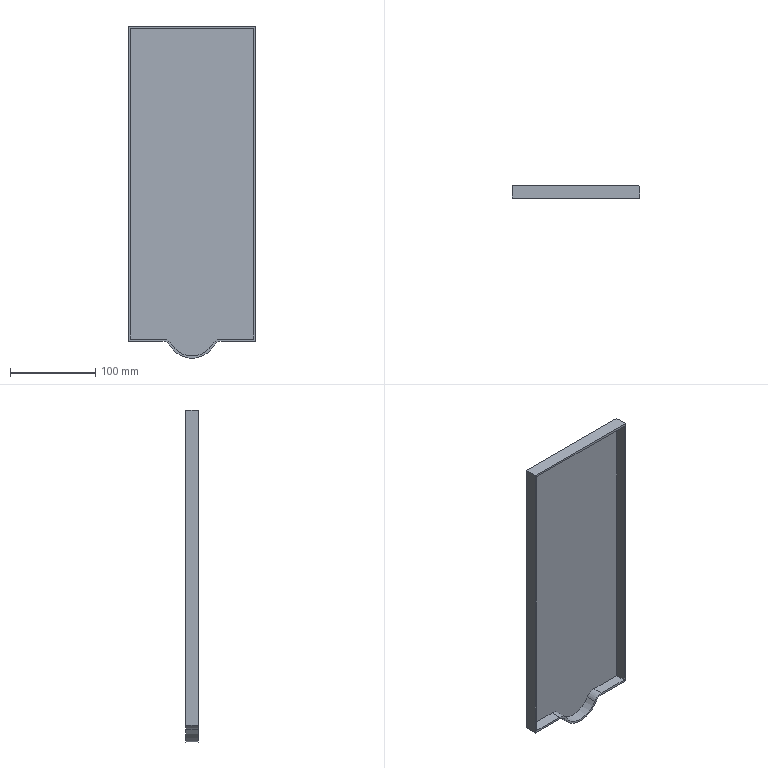Component | SolidWorks | SeedBoxCover-1 | 1 solid | 20 faces | box 150 x 15 x 390 mm | volume 172770 mm3 | plane 13 | cylinder 7 | commonest cylinder face diameters 20 x2 25 x2 60 x1 55 x1 6 x1
build123d program:
from build123d import *

# Parameters (mm, degrees)
SKETCH1_W           = 370
SKETCH1_H           = 150
BOSS_EXTRUDE1_DEPTH = 15
BOSS_EXTRUDE2_DEPTH = 15
FILLET2_R           = 10
SHELL1_T            = -2.5
FILLET3_R           = 3


with BuildPart() as part:
    # Sketch1 → Boss-Extrude1 (new body)
    with BuildSketch(Plane(origin=(0, 0, 0), x_dir=(1, 0, 0), z_dir=(0, 1, 0))):
        Rectangle(SKETCH1_W, SKETCH1_H)
    extrude(amount=BOSS_EXTRUDE1_DEPTH)

    # Sketch3 → Boss-Extrude2 (add)
    with BuildSketch(Plane(origin=(0, 15, 0), x_dir=(1, 0, 0), z_dir=(0, 1, 0))):
        with BuildLine():
            Line((185, 28.284), (185, -28.284))
            ThreePointArc((185, -28.284), (205, 0), (185, 28.284))
        make_face()
    extrude(amount=-BOSS_EXTRUDE2_DEPTH)

    # Fillet2
    fillet2_edges = [part.edges().sort_by_distance(p)[0] for p in [
        (185, 7.5, -28.284),
        (185, 7.5, 28.284),
    ]]
    fillet(fillet2_edges, radius=FILLET2_R)

    # Shell1
    shell1_openings = [part.faces().sort_by_distance(p)[0] for p in [
        (2.873, 0, 0),
    ]]
    offset(amount=SHELL1_T, openings=shell1_openings, kind=Kind.INTERSECTION)

    # Fillet3
    fillet3_edges = [part.edges().sort_by_distance(p)[0] for p in [
        (0, 15, 75),
    ]]
    fillet(fillet3_edges, radius=FILLET3_R)


solid = part.part

# Placed as in the assembly
solid = solid.moved(Location((-5.5, 550, -326.036), (0, 90, 0)))
STEP:
#1=COLOUR_RGB('',0.7922,0.8196,0.9333);
#2=FILL_AREA_STYLE_COLOUR('',#1);
#3=FILL_AREA_STYLE('',(#2));
#4=SURFACE_STYLE_FILL_AREA(#3);
#5=SURFACE_SIDE_STYLE('',(#4));
#6=SURFACE_STYLE_USAGE(.BOTH.,#5);
#7=PRESENTATION_STYLE_ASSIGNMENT((#6));
#8=CARTESIAN_POINT('',(2.736,21.654,-20.12));
#9=VERTEX_POINT('',#8);
#10=CARTESIAN_POINT('',(1.147,21.654,-20.12));
#11=VERTEX_POINT('',#10);
#12=CARTESIAN_POINT('',(2.736,21.654,-20.12));
#13=DIRECTION('',(-1.,-0.,0.));
#14=VECTOR('',#13,39.37);
#15=LINE('',#12,#14);
#16=EDGE_CURVE('',#9,#11,#15,.T.);
#17=ORIENTED_EDGE('',*,*,#16,.F.);
#18=CARTESIAN_POINT('',(2.736,21.654,-5.553));
#19=VERTEX_POINT('',#18);
#20=CARTESIAN_POINT('',(2.736,21.654,-5.553));
#21=DIRECTION('',(-0.,0.,-1.));
#22=VECTOR('',#21,39.37);
#23=LINE('',#20,#22);
#24=EDGE_CURVE('',#19,#9,#23,.T.);
#25=ORIENTED_EDGE('',*,*,#24,.F.);
#26=CARTESIAN_POINT('',(-3.169,21.654,-5.553));
#27=VERTEX_POINT('',#26);
#28=CARTESIAN_POINT('',(2.736,21.654,-5.553));
#29=DIRECTION('',(1.,0.,-0.));
#30=VECTOR('',#29,39.37);
#31=LINE('',#28,#30);
#32=EDGE_CURVE('',#27,#19,#31,.T.);
#33=ORIENTED_EDGE('',*,*,#32,.F.);
#34=CARTESIAN_POINT('',(-3.169,21.654,-20.12));
#35=VERTEX_POINT('',#34);
#36=CARTESIAN_POINT('',(-3.169,21.654,-5.553));
#37=DIRECTION('',(0.,-0.,1.));
#38=VECTOR('',#37,39.37);
#39=LINE('',#36,#38);
#40=EDGE_CURVE('',#35,#27,#39,.T.);
#41=ORIENTED_EDGE('',*,*,#40,.F.);
#42=CARTESIAN_POINT('',(-1.58,21.654,-20.12));
#43=VERTEX_POINT('',#42);
#44=CARTESIAN_POINT('',(2.736,21.654,-20.12));
#45=DIRECTION('',(-1.,-0.,0.));
#46=VECTOR('',#45,39.37);
#47=LINE('',#44,#46);
#48=EDGE_CURVE('',#43,#35,#47,.T.);
#49=ORIENTED_EDGE('',*,*,#48,.F.);
#50=CARTESIAN_POINT('',(-1.239,21.654,-20.316));
#51=VERTEX_POINT('',#50);
#52=CARTESIAN_POINT('',(-1.58,21.654,-20.513));
#53=DIRECTION('',(-0.,1.,0.));
#54=DIRECTION('',(-1.,0.,0.));
#55=AXIS2_PLACEMENT_3D('',#52,#53,#54);
#56=CIRCLE('',#55,0.3937);
#57=EDGE_CURVE('',#43,#51,#56,.T.);
#58=ORIENTED_EDGE('',*,*,#57,.T.);
#59=CARTESIAN_POINT('',(0.8063,21.654,-20.316));
#60=VERTEX_POINT('',#59);
#61=CARTESIAN_POINT('',(-0.2165,21.654,-19.726));
#62=DIRECTION('',(-0.,1.,0.));
#63=DIRECTION('',(-1.,0.,0.));
#64=AXIS2_PLACEMENT_3D('',#61,#62,#63);
#65=CIRCLE('',#64,1.181);
#66=EDGE_CURVE('',#60,#51,#65,.T.);
#67=ORIENTED_EDGE('',*,*,#66,.F.);
#68=CARTESIAN_POINT('',(1.147,21.654,-20.513));
#69=DIRECTION('',(-0.,1.,0.));
#70=DIRECTION('',(-1.,0.,0.));
#71=AXIS2_PLACEMENT_3D('',#68,#69,#70);
#72=CIRCLE('',#71,0.3937);
#73=EDGE_CURVE('',#60,#11,#72,.T.);
#74=ORIENTED_EDGE('',*,*,#73,.T.);
#75=EDGE_LOOP('',(#17,#25,#33,#41,#49,#58,#67,#74));
#76=FACE_OUTER_BOUND('',#75,.T.);
#77=CARTESIAN_POINT('',(2.638,21.654,-5.651));
#78=VERTEX_POINT('',#77);
#79=CARTESIAN_POINT('',(2.638,21.654,-20.021));
#80=VERTEX_POINT('',#79);
#81=CARTESIAN_POINT('',(2.638,21.654,-12.836));
#82=DIRECTION('',(-0.,0.,-1.));
#83=VECTOR('',#82,39.37);
#84=LINE('',#81,#83);
#85=EDGE_CURVE('',#78,#80,#84,.T.);
#86=ORIENTED_EDGE('',*,*,#85,.T.);
#87=CARTESIAN_POINT('',(1.147,21.654,-20.021));
#88=VERTEX_POINT('',#87);
#89=CARTESIAN_POINT('',(-0.2165,21.654,-20.021));
#90=DIRECTION('',(-1.,-0.,0.));
#91=VECTOR('',#90,39.37);
#92=LINE('',#89,#91);
#93=EDGE_CURVE('',#80,#88,#92,.T.);
#94=ORIENTED_EDGE('',*,*,#93,.T.);
#95=CARTESIAN_POINT('',(0.7211,21.654,-20.267));
#96=VERTEX_POINT('',#95);
#97=CARTESIAN_POINT('',(1.147,21.654,-20.513));
#98=DIRECTION('',(-0.,1.,0.));
#99=DIRECTION('',(-1.,0.,0.));
#100=AXIS2_PLACEMENT_3D('',#97,#98,#99);
#101=CIRCLE('',#100,0.4921);
#102=EDGE_CURVE('',#96,#88,#101,.T.);
#103=ORIENTED_EDGE('',*,*,#102,.F.);
#104=CARTESIAN_POINT('',(-1.154,21.654,-20.267));
#105=VERTEX_POINT('',#104);
#106=CARTESIAN_POINT('',(-0.2165,21.654,-19.726));
#107=DIRECTION('',(-0.,1.,0.));
#108=DIRECTION('',(-1.,0.,-0.));
#109=AXIS2_PLACEMENT_3D('',#106,#107,#108);
#110=CIRCLE('',#109,1.083);
#111=EDGE_CURVE('',#96,#105,#110,.T.);
#112=ORIENTED_EDGE('',*,*,#111,.T.);
#113=CARTESIAN_POINT('',(-1.58,21.654,-20.021));
#114=VERTEX_POINT('',#113);
#115=CARTESIAN_POINT('',(-1.58,21.654,-20.513));
#116=DIRECTION('',(-0.,1.,0.));
#117=DIRECTION('',(-1.,0.,0.));
#118=AXIS2_PLACEMENT_3D('',#115,#116,#117);
#119=CIRCLE('',#118,0.4921);
#120=EDGE_CURVE('',#114,#105,#119,.T.);
#121=ORIENTED_EDGE('',*,*,#120,.F.);
#122=CARTESIAN_POINT('',(-3.071,21.654,-20.021));
#123=VERTEX_POINT('',#122);
#124=CARTESIAN_POINT('',(-0.2165,21.654,-20.021));
#125=DIRECTION('',(-1.,-0.,0.));
#126=VECTOR('',#125,39.37);
#127=LINE('',#124,#126);
#128=EDGE_CURVE('',#114,#123,#127,.T.);
#129=ORIENTED_EDGE('',*,*,#128,.T.);
#130=CARTESIAN_POINT('',(-3.071,21.654,-5.651));
#131=VERTEX_POINT('',#130);
#132=CARTESIAN_POINT('',(-3.071,21.654,-12.836));
#133=DIRECTION('',(0.,-0.,1.));
#134=VECTOR('',#133,39.37);
#135=LINE('',#132,#134);
#136=EDGE_CURVE('',#123,#131,#135,.T.);
#137=ORIENTED_EDGE('',*,*,#136,.T.);
#138=CARTESIAN_POINT('',(-0.2165,21.654,-5.651));
#139=DIRECTION('',(1.,0.,-0.));
#140=VECTOR('',#139,39.37);
#141=LINE('',#138,#140);
#142=EDGE_CURVE('',#131,#78,#141,.T.);
#143=ORIENTED_EDGE('',*,*,#142,.T.);
#144=EDGE_LOOP('',(#86,#94,#103,#112,#121,#129,#137,#143));
#145=FACE_BOUND('',#144,.T.);
#146=CARTESIAN_POINT('',(-0.2165,21.654,-12.836));
#147=DIRECTION('',(0.,-1.,-0.));
#148=DIRECTION('',(-1.,-0.,0.));
#149=AXIS2_PLACEMENT_3D('',#146,#147,#148);
#150=PLANE('',#149);
#151=ADVANCED_FACE('',(#76,#145),#150,.T.);
#152=CARTESIAN_POINT('',(2.618,22.244,-20.12));
#153=VERTEX_POINT('',#152);
#154=CARTESIAN_POINT('',(1.147,22.244,-20.12));
#155=VERTEX_POINT('',#154);
#156=CARTESIAN_POINT('',(2.736,22.244,-20.12));
#157=DIRECTION('',(-1.,-0.,0.));
#158=VECTOR('',#157,39.37);
#159=LINE('',#156,#158);
#160=EDGE_CURVE('',#153,#155,#159,.T.);
#161=ORIENTED_EDGE('',*,*,#160,.F.);
#162=CARTESIAN_POINT('',(2.736,22.126,-20.12));
#163=VERTEX_POINT('',#162);
#164=CARTESIAN_POINT('',(2.618,22.126,-20.12));
#165=DIRECTION('',(-0.,0.,-1.));
#166=DIRECTION('',(1.,0.,0.));
#167=AXIS2_PLACEMENT_3D('',#164,#165,#166);
#168=CIRCLE('',#167,0.1181);
#169=EDGE_CURVE('',#153,#163,#168,.T.);
#170=ORIENTED_EDGE('',*,*,#169,.T.);
#171=CARTESIAN_POINT('',(2.736,22.244,-20.12));
#172=DIRECTION('',(0.,-1.,-0.));
#173=VECTOR('',#172,39.37);
#174=LINE('',#171,#173);
#175=EDGE_CURVE('',#163,#9,#174,.T.);
#176=ORIENTED_EDGE('',*,*,#175,.T.);
#177=ORIENTED_EDGE('',*,*,#16,.T.);
#178=CARTESIAN_POINT('',(1.147,22.244,-20.12));
#179=DIRECTION('',(-0.,1.,0.));
#180=VECTOR('',#179,39.37);
#181=LINE('',#178,#180);
#182=EDGE_CURVE('',#11,#155,#181,.T.);
#183=ORIENTED_EDGE('',*,*,#182,.T.);
#184=EDGE_LOOP('',(#161,#170,#176,#177,#183));
#185=FACE_OUTER_BOUND('',#184,.T.);
#186=CARTESIAN_POINT('',(2.736,22.244,-20.12));
#187=DIRECTION('',(0.,-0.,1.));
#188=DIRECTION('',(1.,0.,-0.));
#189=AXIS2_PLACEMENT_3D('',#186,#187,#188);
#190=PLANE('',#189);
#191=ADVANCED_FACE('',(#185),#190,.F.);
#192=CARTESIAN_POINT('',(-1.58,22.244,-20.12));
#193=VERTEX_POINT('',#192);
#194=CARTESIAN_POINT('',(-3.169,22.244,-20.12));
#195=VERTEX_POINT('',#194);
#196=CARTESIAN_POINT('',(2.736,22.244,-20.12));
#197=DIRECTION('',(-1.,-0.,0.));
#198=VECTOR('',#197,39.37);
#199=LINE('',#196,#198);
#200=EDGE_CURVE('',#193,#195,#199,.T.);
#201=ORIENTED_EDGE('',*,*,#200,.F.);
#202=CARTESIAN_POINT('',(-1.58,22.244,-20.12));
#203=DIRECTION('',(0.,-1.,-0.));
#204=VECTOR('',#203,39.37);
#205=LINE('',#202,#204);
#206=EDGE_CURVE('',#193,#43,#205,.T.);
#207=ORIENTED_EDGE('',*,*,#206,.T.);
#208=ORIENTED_EDGE('',*,*,#48,.T.);
#209=CARTESIAN_POINT('',(-3.169,22.244,-20.12));
#210=DIRECTION('',(0.,-1.,-0.));
#211=VECTOR('',#210,39.37);
#212=LINE('',#209,#211);
#213=EDGE_CURVE('',#195,#35,#212,.T.);
#214=ORIENTED_EDGE('',*,*,#213,.F.);
#215=EDGE_LOOP('',(#201,#207,#208,#214));
#216=FACE_OUTER_BOUND('',#215,.T.);
#217=CARTESIAN_POINT('',(2.736,22.244,-20.12));
#218=DIRECTION('',(0.,-0.,1.));
#219=DIRECTION('',(1.,0.,-0.));
#220=AXIS2_PLACEMENT_3D('',#217,#218,#219);
#221=PLANE('',#220);
#222=ADVANCED_FACE('',(#216),#221,.F.);
#223=ORIENTED_EDGE('',*,*,#40,.T.);
#224=CARTESIAN_POINT('',(-3.169,22.244,-5.553));
#225=VERTEX_POINT('',#224);
#226=CARTESIAN_POINT('',(-3.169,22.244,-5.553));
#227=DIRECTION('',(0.,-1.,-0.));
#228=VECTOR('',#227,39.37);
#229=LINE('',#226,#228);
#230=EDGE_CURVE('',#225,#27,#229,.T.);
#231=ORIENTED_EDGE('',*,*,#230,.F.);
#232=CARTESIAN_POINT('',(-3.169,22.244,-5.553));
#233=DIRECTION('',(0.,-0.,1.));
#234=VECTOR('',#233,39.37);
#235=LINE('',#232,#234);
#236=EDGE_CURVE('',#195,#225,#235,.T.);
#237=ORIENTED_EDGE('',*,*,#236,.F.);
#238=ORIENTED_EDGE('',*,*,#213,.T.);
#239=EDGE_LOOP('',(#223,#231,#237,#238));
#240=FACE_OUTER_BOUND('',#239,.T.);
#241=CARTESIAN_POINT('',(-3.169,22.244,-5.553));
#242=DIRECTION('',(1.,0.,-0.));
#243=DIRECTION('',(-0.,0.,-1.));
#244=AXIS2_PLACEMENT_3D('',#241,#242,#243);
#245=PLANE('',#244);
#246=ADVANCED_FACE('',(#240),#245,.F.);
#247=CARTESIAN_POINT('',(2.736,22.126,-5.553));
#248=VERTEX_POINT('',#247);
#249=CARTESIAN_POINT('',(2.736,22.244,-5.553));
#250=DIRECTION('',(0.,-1.,-0.));
#251=VECTOR('',#250,39.37);
#252=LINE('',#249,#251);
#253=EDGE_CURVE('',#248,#19,#252,.T.);
#254=ORIENTED_EDGE('',*,*,#253,.F.);
#255=CARTESIAN_POINT('',(2.618,22.244,-5.553));
#256=VERTEX_POINT('',#255);
#257=CARTESIAN_POINT('',(2.618,22.126,-5.553));
#258=DIRECTION('',(0.,-0.,1.));
#259=DIRECTION('',(-1.,0.,0.));
#260=AXIS2_PLACEMENT_3D('',#257,#258,#259);
#261=CIRCLE('',#260,0.1181);
#262=EDGE_CURVE('',#248,#256,#261,.T.);
#263=ORIENTED_EDGE('',*,*,#262,.T.);
#264=CARTESIAN_POINT('',(2.736,22.244,-5.553));
#265=DIRECTION('',(1.,0.,-0.));
#266=VECTOR('',#265,39.37);
#267=LINE('',#264,#266);
#268=EDGE_CURVE('',#225,#256,#267,.T.);
#269=ORIENTED_EDGE('',*,*,#268,.F.);
#270=ORIENTED_EDGE('',*,*,#230,.T.);
#271=ORIENTED_EDGE('',*,*,#32,.T.);
#272=EDGE_LOOP('',(#254,#263,#269,#270,#271));
#273=FACE_OUTER_BOUND('',#272,.T.);
#274=CARTESIAN_POINT('',(2.736,22.244,-5.553));
#275=DIRECTION('',(-0.,0.,-1.));
#276=DIRECTION('',(-1.,-0.,0.));
#277=AXIS2_PLACEMENT_3D('',#274,#275,#276);
#278=PLANE('',#277);
#279=ADVANCED_FACE('',(#273),#278,.F.);
#280=ORIENTED_EDGE('',*,*,#175,.F.);
#281=CARTESIAN_POINT('',(2.736,22.126,-5.553));
#282=DIRECTION('',(0.,-0.,1.));
#283=VECTOR('',#282,39.37);
#284=LINE('',#281,#283);
#285=EDGE_CURVE('',#163,#248,#284,.T.);
#286=ORIENTED_EDGE('',*,*,#285,.T.);
#287=ORIENTED_EDGE('',*,*,#253,.T.);
#288=ORIENTED_EDGE('',*,*,#24,.T.);
#289=EDGE_LOOP('',(#280,#286,#287,#288));
#290=FACE_OUTER_BOUND('',#289,.T.);
#291=CARTESIAN_POINT('',(2.736,22.244,-5.553));
#292=DIRECTION('',(-1.,-0.,0.));
#293=DIRECTION('',(0.,-0.,1.));
#294=AXIS2_PLACEMENT_3D('',#291,#292,#293);
#295=PLANE('',#294);
#296=ADVANCED_FACE('',(#290),#295,.F.);
#297=ORIENTED_EDGE('',*,*,#268,.T.);
#298=CARTESIAN_POINT('',(2.618,22.244,-12.836));
#299=DIRECTION('',(-0.,0.,-1.));
#300=VECTOR('',#299,39.37);
#301=LINE('',#298,#300);
#302=EDGE_CURVE('',#256,#153,#301,.T.);
#303=ORIENTED_EDGE('',*,*,#302,.T.);
#304=ORIENTED_EDGE('',*,*,#160,.T.);
#305=CARTESIAN_POINT('',(0.8063,22.244,-20.316));
#306=VERTEX_POINT('',#305);
#307=CARTESIAN_POINT('',(1.147,22.244,-20.513));
#308=DIRECTION('',(0.,-1.,-0.));
#309=DIRECTION('',(-1.,0.,0.));
#310=AXIS2_PLACEMENT_3D('',#307,#308,#309);
#311=CIRCLE('',#310,0.3937);
#312=EDGE_CURVE('',#155,#306,#311,.T.);
#313=ORIENTED_EDGE('',*,*,#312,.T.);
#314=CARTESIAN_POINT('',(-1.239,22.244,-20.316));
#315=VERTEX_POINT('',#314);
#316=CARTESIAN_POINT('',(-0.2165,22.244,-19.726));
#317=DIRECTION('',(-0.,1.,0.));
#318=DIRECTION('',(-1.,0.,0.));
#319=AXIS2_PLACEMENT_3D('',#316,#317,#318);
#320=CIRCLE('',#319,1.181);
#321=EDGE_CURVE('',#306,#315,#320,.T.);
#322=ORIENTED_EDGE('',*,*,#321,.T.);
#323=CARTESIAN_POINT('',(-1.58,22.244,-20.513));
#324=DIRECTION('',(0.,-1.,-0.));
#325=DIRECTION('',(-1.,0.,0.));
#326=AXIS2_PLACEMENT_3D('',#323,#324,#325);
#327=CIRCLE('',#326,0.3937);
#328=EDGE_CURVE('',#315,#193,#327,.T.);
#329=ORIENTED_EDGE('',*,*,#328,.T.);
#330=ORIENTED_EDGE('',*,*,#200,.T.);
#331=ORIENTED_EDGE('',*,*,#236,.T.);
#332=EDGE_LOOP('',(#297,#303,#304,#313,#322,#329,#330,#331));
#333=FACE_OUTER_BOUND('',#332,.T.);
#334=CARTESIAN_POINT('',(-0.2165,22.244,-12.836));
#335=DIRECTION('',(0.,-1.,-0.));
#336=DIRECTION('',(-1.,-0.,0.));
#337=AXIS2_PLACEMENT_3D('',#334,#335,#336);
#338=PLANE('',#337);
#339=ADVANCED_FACE('',(#333),#338,.F.);
#340=ORIENTED_EDGE('',*,*,#321,.F.);
#341=CARTESIAN_POINT('',(0.8063,21.654,-20.316));
#342=DIRECTION('',(0.,-1.,-0.));
#343=VECTOR('',#342,39.37);
#344=LINE('',#341,#343);
#345=EDGE_CURVE('',#306,#60,#344,.T.);
#346=ORIENTED_EDGE('',*,*,#345,.T.);
#347=ORIENTED_EDGE('',*,*,#66,.T.);
#348=CARTESIAN_POINT('',(-1.239,21.654,-20.316));
#349=DIRECTION('',(-0.,1.,0.));
#350=VECTOR('',#349,39.37);
#351=LINE('',#348,#350);
#352=EDGE_CURVE('',#51,#315,#351,.T.);
#353=ORIENTED_EDGE('',*,*,#352,.T.);
#354=EDGE_LOOP('',(#340,#346,#347,#353));
#355=FACE_OUTER_BOUND('',#354,.T.);
#356=CARTESIAN_POINT('',(-0.2165,21.654,-19.726));
#357=DIRECTION('',(-0.,1.,0.));
#358=DIRECTION('',(1.,0.,0.));
#359=AXIS2_PLACEMENT_3D('',#356,#357,#358);
#360=CYLINDRICAL_SURFACE('',#359,1.181);
#361=ADVANCED_FACE('',(#355),#360,.T.);
#362=ORIENTED_EDGE('',*,*,#73,.F.);
#363=ORIENTED_EDGE('',*,*,#345,.F.);
#364=ORIENTED_EDGE('',*,*,#312,.F.);
#365=ORIENTED_EDGE('',*,*,#182,.F.);
#366=EDGE_LOOP('',(#362,#363,#364,#365));
#367=FACE_OUTER_BOUND('',#366,.T.);
#368=CARTESIAN_POINT('',(1.147,21.654,-20.513));
#369=DIRECTION('',(-0.,1.,0.));
#370=DIRECTION('',(1.,0.,0.));
#371=AXIS2_PLACEMENT_3D('',#368,#369,#370);
#372=CYLINDRICAL_SURFACE('',#371,0.3937);
#373=ADVANCED_FACE('',(#367),#372,.F.);
#374=ORIENTED_EDGE('',*,*,#57,.F.);
#375=ORIENTED_EDGE('',*,*,#206,.F.);
#376=ORIENTED_EDGE('',*,*,#328,.F.);
#377=ORIENTED_EDGE('',*,*,#352,.F.);
#378=EDGE_LOOP('',(#374,#375,#376,#377));
#379=FACE_OUTER_BOUND('',#378,.T.);
#380=CARTESIAN_POINT('',(-1.58,21.654,-20.513));
#381=DIRECTION('',(-0.,1.,0.));
#382=DIRECTION('',(1.,0.,0.));
#383=AXIS2_PLACEMENT_3D('',#380,#381,#382);
#384=CYLINDRICAL_SURFACE('',#383,0.3937);
#385=ADVANCED_FACE('',(#379),#384,.F.);
#386=ORIENTED_EDGE('',*,*,#93,.F.);
#387=CARTESIAN_POINT('',(2.638,22.146,-20.021));
#388=VERTEX_POINT('',#387);
#389=CARTESIAN_POINT('',(2.638,22.244,-20.021));
#390=DIRECTION('',(0.,-1.,-0.));
#391=VECTOR('',#390,39.37);
#392=LINE('',#389,#391);
#393=EDGE_CURVE('',#388,#80,#392,.T.);
#394=ORIENTED_EDGE('',*,*,#393,.F.);
#395=CARTESIAN_POINT('',(1.147,22.146,-20.021));
#396=VERTEX_POINT('',#395);
#397=CARTESIAN_POINT('',(-0.2165,22.146,-20.021));
#398=DIRECTION('',(-1.,-0.,0.));
#399=VECTOR('',#398,39.37);
#400=LINE('',#397,#399);
#401=EDGE_CURVE('',#388,#396,#400,.T.);
#402=ORIENTED_EDGE('',*,*,#401,.T.);
#403=CARTESIAN_POINT('',(1.147,22.244,-20.021));
#404=DIRECTION('',(-0.,1.,0.));
#405=VECTOR('',#404,39.37);
#406=LINE('',#403,#405);
#407=EDGE_CURVE('',#88,#396,#406,.T.);
#408=ORIENTED_EDGE('',*,*,#407,.F.);
#409=EDGE_LOOP('',(#386,#394,#402,#408));
#410=FACE_OUTER_BOUND('',#409,.T.);
#411=CARTESIAN_POINT('',(2.736,22.244,-20.021));
#412=DIRECTION('',(0.,-0.,1.));
#413=DIRECTION('',(1.,0.,-0.));
#414=AXIS2_PLACEMENT_3D('',#411,#412,#413);
#415=PLANE('',#414);
#416=ADVANCED_FACE('',(#410),#415,.T.);
#417=CARTESIAN_POINT('',(-1.58,22.146,-20.021));
#418=VERTEX_POINT('',#417);
#419=CARTESIAN_POINT('',(-3.071,22.146,-20.021));
#420=VERTEX_POINT('',#419);
#421=CARTESIAN_POINT('',(-0.2165,22.146,-20.021));
#422=DIRECTION('',(-1.,-0.,0.));
#423=VECTOR('',#422,39.37);
#424=LINE('',#421,#423);
#425=EDGE_CURVE('',#418,#420,#424,.T.);
#426=ORIENTED_EDGE('',*,*,#425,.T.);
#427=CARTESIAN_POINT('',(-3.071,22.244,-20.021));
#428=DIRECTION('',(0.,-1.,-0.));
#429=VECTOR('',#428,39.37);
#430=LINE('',#427,#429);
#431=EDGE_CURVE('',#420,#123,#430,.T.);
#432=ORIENTED_EDGE('',*,*,#431,.T.);
#433=ORIENTED_EDGE('',*,*,#128,.F.);
#434=CARTESIAN_POINT('',(-1.58,22.244,-20.021));
#435=DIRECTION('',(0.,-1.,-0.));
#436=VECTOR('',#435,39.37);
#437=LINE('',#434,#436);
#438=EDGE_CURVE('',#418,#114,#437,.T.);
#439=ORIENTED_EDGE('',*,*,#438,.F.);
#440=EDGE_LOOP('',(#426,#432,#433,#439));
#441=FACE_OUTER_BOUND('',#440,.T.);
#442=CARTESIAN_POINT('',(2.736,22.244,-20.021));
#443=DIRECTION('',(0.,-0.,1.));
#444=DIRECTION('',(1.,0.,-0.));
#445=AXIS2_PLACEMENT_3D('',#442,#443,#444);
#446=PLANE('',#445);
#447=ADVANCED_FACE('',(#441),#446,.T.);
#448=ORIENTED_EDGE('',*,*,#136,.F.);
#449=ORIENTED_EDGE('',*,*,#431,.F.);
#450=CARTESIAN_POINT('',(-3.071,22.146,-5.651));
#451=VERTEX_POINT('',#450);
#452=CARTESIAN_POINT('',(-3.071,22.146,-12.836));
#453=DIRECTION('',(0.,-0.,1.));
#454=VECTOR('',#453,39.37);
#455=LINE('',#452,#454);
#456=EDGE_CURVE('',#420,#451,#455,.T.);
#457=ORIENTED_EDGE('',*,*,#456,.T.);
#458=CARTESIAN_POINT('',(-3.071,22.244,-5.651));
#459=DIRECTION('',(0.,-1.,-0.));
#460=VECTOR('',#459,39.37);
#461=LINE('',#458,#460);
#462=EDGE_CURVE('',#451,#131,#461,.T.);
#463=ORIENTED_EDGE('',*,*,#462,.T.);
#464=EDGE_LOOP('',(#448,#449,#457,#463));
#465=FACE_OUTER_BOUND('',#464,.T.);
#466=CARTESIAN_POINT('',(-3.071,22.244,-5.553));
#467=DIRECTION('',(1.,0.,-0.));
#468=DIRECTION('',(-0.,0.,-1.));
#469=AXIS2_PLACEMENT_3D('',#466,#467,#468);
#470=PLANE('',#469);
#471=ADVANCED_FACE('',(#465),#470,.T.);
#472=ORIENTED_EDGE('',*,*,#142,.F.);
#473=ORIENTED_EDGE('',*,*,#462,.F.);
#474=CARTESIAN_POINT('',(2.638,22.146,-5.651));
#475=VERTEX_POINT('',#474);
#476=CARTESIAN_POINT('',(-0.2165,22.146,-5.651));
#477=DIRECTION('',(1.,0.,-0.));
#478=VECTOR('',#477,39.37);
#479=LINE('',#476,#478);
#480=EDGE_CURVE('',#451,#475,#479,.T.);
#481=ORIENTED_EDGE('',*,*,#480,.T.);
#482=CARTESIAN_POINT('',(2.638,22.244,-5.651));
#483=DIRECTION('',(0.,-1.,-0.));
#484=VECTOR('',#483,39.37);
#485=LINE('',#482,#484);
#486=EDGE_CURVE('',#475,#78,#485,.T.);
#487=ORIENTED_EDGE('',*,*,#486,.T.);
#488=EDGE_LOOP('',(#472,#473,#481,#487));
#489=FACE_OUTER_BOUND('',#488,.T.);
#490=CARTESIAN_POINT('',(2.736,22.244,-5.651));
#491=DIRECTION('',(-0.,0.,-1.));
#492=DIRECTION('',(-1.,-0.,0.));
#493=AXIS2_PLACEMENT_3D('',#490,#491,#492);
#494=PLANE('',#493);
#495=ADVANCED_FACE('',(#489),#494,.T.);
#496=ORIENTED_EDGE('',*,*,#85,.F.);
#497=ORIENTED_EDGE('',*,*,#486,.F.);
#498=CARTESIAN_POINT('',(2.638,22.146,-12.836));
#499=DIRECTION('',(-0.,0.,-1.));
#500=VECTOR('',#499,39.37);
#501=LINE('',#498,#500);
#502=EDGE_CURVE('',#475,#388,#501,.T.);
#503=ORIENTED_EDGE('',*,*,#502,.T.);
#504=ORIENTED_EDGE('',*,*,#393,.T.);
#505=EDGE_LOOP('',(#496,#497,#503,#504));
#506=FACE_OUTER_BOUND('',#505,.T.);
#507=CARTESIAN_POINT('',(2.638,22.244,-5.553));
#508=DIRECTION('',(-1.,-0.,0.));
#509=DIRECTION('',(0.,-0.,1.));
#510=AXIS2_PLACEMENT_3D('',#507,#508,#509);
#511=PLANE('',#510);
#512=ADVANCED_FACE('',(#506),#511,.T.);
#513=ORIENTED_EDGE('',*,*,#401,.F.);
#514=ORIENTED_EDGE('',*,*,#502,.F.);
#515=ORIENTED_EDGE('',*,*,#480,.F.);
#516=ORIENTED_EDGE('',*,*,#456,.F.);
#517=ORIENTED_EDGE('',*,*,#425,.F.);
#518=CARTESIAN_POINT('',(-1.154,22.146,-20.267));
#519=VERTEX_POINT('',#518);
#520=CARTESIAN_POINT('',(-1.58,22.146,-20.513));
#521=DIRECTION('',(0.,-1.,-0.));
#522=DIRECTION('',(-1.,0.,0.));
#523=AXIS2_PLACEMENT_3D('',#520,#521,#522);
#524=CIRCLE('',#523,0.4921);
#525=EDGE_CURVE('',#519,#418,#524,.T.);
#526=ORIENTED_EDGE('',*,*,#525,.F.);
#527=CARTESIAN_POINT('',(0.7211,22.146,-20.267));
#528=VERTEX_POINT('',#527);
#529=CARTESIAN_POINT('',(-0.2165,22.146,-19.726));
#530=DIRECTION('',(-0.,1.,0.));
#531=DIRECTION('',(-1.,0.,-0.));
#532=AXIS2_PLACEMENT_3D('',#529,#530,#531);
#533=CIRCLE('',#532,1.083);
#534=EDGE_CURVE('',#528,#519,#533,.T.);
#535=ORIENTED_EDGE('',*,*,#534,.F.);
#536=CARTESIAN_POINT('',(1.147,22.146,-20.513));
#537=DIRECTION('',(0.,-1.,-0.));
#538=DIRECTION('',(-1.,0.,0.));
#539=AXIS2_PLACEMENT_3D('',#536,#537,#538);
#540=CIRCLE('',#539,0.4921);
#541=EDGE_CURVE('',#396,#528,#540,.T.);
#542=ORIENTED_EDGE('',*,*,#541,.F.);
#543=EDGE_LOOP('',(#513,#514,#515,#516,#517,#526,#535,#542));
#544=FACE_OUTER_BOUND('',#543,.T.);
#545=CARTESIAN_POINT('',(-0.2165,22.146,-12.836));
#546=DIRECTION('',(0.,-1.,-0.));
#547=DIRECTION('',(-1.,-0.,0.));
#548=AXIS2_PLACEMENT_3D('',#545,#546,#547);
#549=PLANE('',#548);
#550=ADVANCED_FACE('',(#544),#549,.T.);
#551=ORIENTED_EDGE('',*,*,#534,.T.);
#552=CARTESIAN_POINT('',(-1.154,21.654,-20.267));
#553=DIRECTION('',(-0.,1.,0.));
#554=VECTOR('',#553,39.37);
#555=LINE('',#552,#554);
#556=EDGE_CURVE('',#105,#519,#555,.T.);
#557=ORIENTED_EDGE('',*,*,#556,.F.);
#558=ORIENTED_EDGE('',*,*,#111,.F.);
#559=CARTESIAN_POINT('',(0.7211,21.654,-20.267));
#560=DIRECTION('',(0.,-1.,-0.));
#561=VECTOR('',#560,39.37);
#562=LINE('',#559,#561);
#563=EDGE_CURVE('',#528,#96,#562,.T.);
#564=ORIENTED_EDGE('',*,*,#563,.F.);
#565=EDGE_LOOP('',(#551,#557,#558,#564));
#566=FACE_OUTER_BOUND('',#565,.T.);
#567=CARTESIAN_POINT('',(-0.2165,21.654,-19.726));
#568=DIRECTION('',(-0.,1.,0.));
#569=DIRECTION('',(1.,0.,0.));
#570=AXIS2_PLACEMENT_3D('',#567,#568,#569);
#571=CYLINDRICAL_SURFACE('',#570,1.083);
#572=ADVANCED_FACE('',(#566),#571,.F.);
#573=ORIENTED_EDGE('',*,*,#102,.T.);
#574=ORIENTED_EDGE('',*,*,#407,.T.);
#575=ORIENTED_EDGE('',*,*,#541,.T.);
#576=ORIENTED_EDGE('',*,*,#563,.T.);
#577=EDGE_LOOP('',(#573,#574,#575,#576));
#578=FACE_OUTER_BOUND('',#577,.T.);
#579=CARTESIAN_POINT('',(1.147,21.654,-20.513));
#580=DIRECTION('',(-0.,1.,0.));
#581=DIRECTION('',(1.,0.,0.));
#582=AXIS2_PLACEMENT_3D('',#579,#580,#581);
#583=CYLINDRICAL_SURFACE('',#582,0.4921);
#584=ADVANCED_FACE('',(#578),#583,.T.);
#585=ORIENTED_EDGE('',*,*,#120,.T.);
#586=ORIENTED_EDGE('',*,*,#556,.T.);
#587=ORIENTED_EDGE('',*,*,#525,.T.);
#588=ORIENTED_EDGE('',*,*,#438,.T.);
#589=EDGE_LOOP('',(#585,#586,#587,#588));
#590=FACE_OUTER_BOUND('',#589,.T.);
#591=CARTESIAN_POINT('',(-1.58,21.654,-20.513));
#592=DIRECTION('',(-0.,1.,0.));
#593=DIRECTION('',(1.,0.,0.));
#594=AXIS2_PLACEMENT_3D('',#591,#592,#593);
#595=CYLINDRICAL_SURFACE('',#594,0.4921);
#596=ADVANCED_FACE('',(#590),#595,.T.);
#597=ORIENTED_EDGE('',*,*,#262,.F.);
#598=ORIENTED_EDGE('',*,*,#285,.F.);
#599=ORIENTED_EDGE('',*,*,#169,.F.);
#600=ORIENTED_EDGE('',*,*,#302,.F.);
#601=EDGE_LOOP('',(#597,#598,#599,#600));
#602=FACE_OUTER_BOUND('',#601,.T.);
#603=CARTESIAN_POINT('',(2.618,22.126,-12.836));
#604=DIRECTION('',(-0.,0.,-1.));
#605=DIRECTION('',(-1.,0.,0.));
#606=AXIS2_PLACEMENT_3D('',#603,#604,#605);
#607=CYLINDRICAL_SURFACE('',#606,0.1181);
#608=ADVANCED_FACE('',(#602),#607,.T.);
#609=CLOSED_SHELL('',(#151,#191,#222,#246,#279,#296,#339,#361,#373,#385,#416,#447,#471,#495,#512,#550,#572,#584,#596,#608));
#610=MANIFOLD_SOLID_BREP('',#609);
#611=STYLED_ITEM('',(#7),#610);
#612=PRESENTATION_LAYER_ASSIGNMENT('','',(#611));
#613=CARTESIAN_POINT('',(0.,0.,0.));
#614=DIRECTION('',(0.,0.,1.));
#615=DIRECTION('',(1.,0.,0.));
#616=AXIS2_PLACEMENT_3D('',#613,#614,#615);
#617=(LENGTH_UNIT()NAMED_UNIT(*)SI_UNIT($,.METRE.));
#618=LENGTH_MEASURE_WITH_UNIT(LENGTH_MEASURE(0.0254),#617);
#619=DIMENSIONAL_EXPONENTS(1.,0.,0.,0.,0.,0.,0.);
#620=(CONVERSION_BASED_UNIT('',#618)LENGTH_UNIT()NAMED_UNIT(#619));
#621=UNCERTAINTY_MEASURE_WITH_UNIT(LENGTH_MEASURE(0.00001),#620,'','');
#622=(NAMED_UNIT(*)PLANE_ANGLE_UNIT()SI_UNIT($,.RADIAN.));
#623=(NAMED_UNIT(*)SI_UNIT($,.STERADIAN.)SOLID_ANGLE_UNIT());
#624=(GEOMETRIC_REPRESENTATION_CONTEXT(3)GLOBAL_UNCERTAINTY_ASSIGNED_CONTEXT((#621))GLOBAL_UNIT_ASSIGNED_CONTEXT((#620,#622,#623))REPRESENTATION_CONTEXT('',''));
#625=ADVANCED_BREP_SHAPE_REPRESENTATION('',(#610,#616),#624);
#626=(LENGTH_UNIT()NAMED_UNIT(*)SI_UNIT($,.METRE.));
#627=LENGTH_MEASURE_WITH_UNIT(LENGTH_MEASURE(0.0254),#626);
#628=DIMENSIONAL_EXPONENTS(1.,0.,0.,0.,0.,0.,0.);
#629=(CONVERSION_BASED_UNIT('',#627)LENGTH_UNIT()NAMED_UNIT(#628));
#630=UNCERTAINTY_MEASURE_WITH_UNIT(LENGTH_MEASURE(0.00001),#629,'','');
#631=(NAMED_UNIT(*)PLANE_ANGLE_UNIT()SI_UNIT($,.RADIAN.));
#632=(NAMED_UNIT(*)SI_UNIT($,.STERADIAN.)SOLID_ANGLE_UNIT());
#633=(GEOMETRIC_REPRESENTATION_CONTEXT(3)GLOBAL_UNCERTAINTY_ASSIGNED_CONTEXT((#630))GLOBAL_UNIT_ASSIGNED_CONTEXT((#629,#631,#632))REPRESENTATION_CONTEXT('',''));
#634=MECHANICAL_DESIGN_GEOMETRIC_PRESENTATION_REPRESENTATION('',(#611),#633);